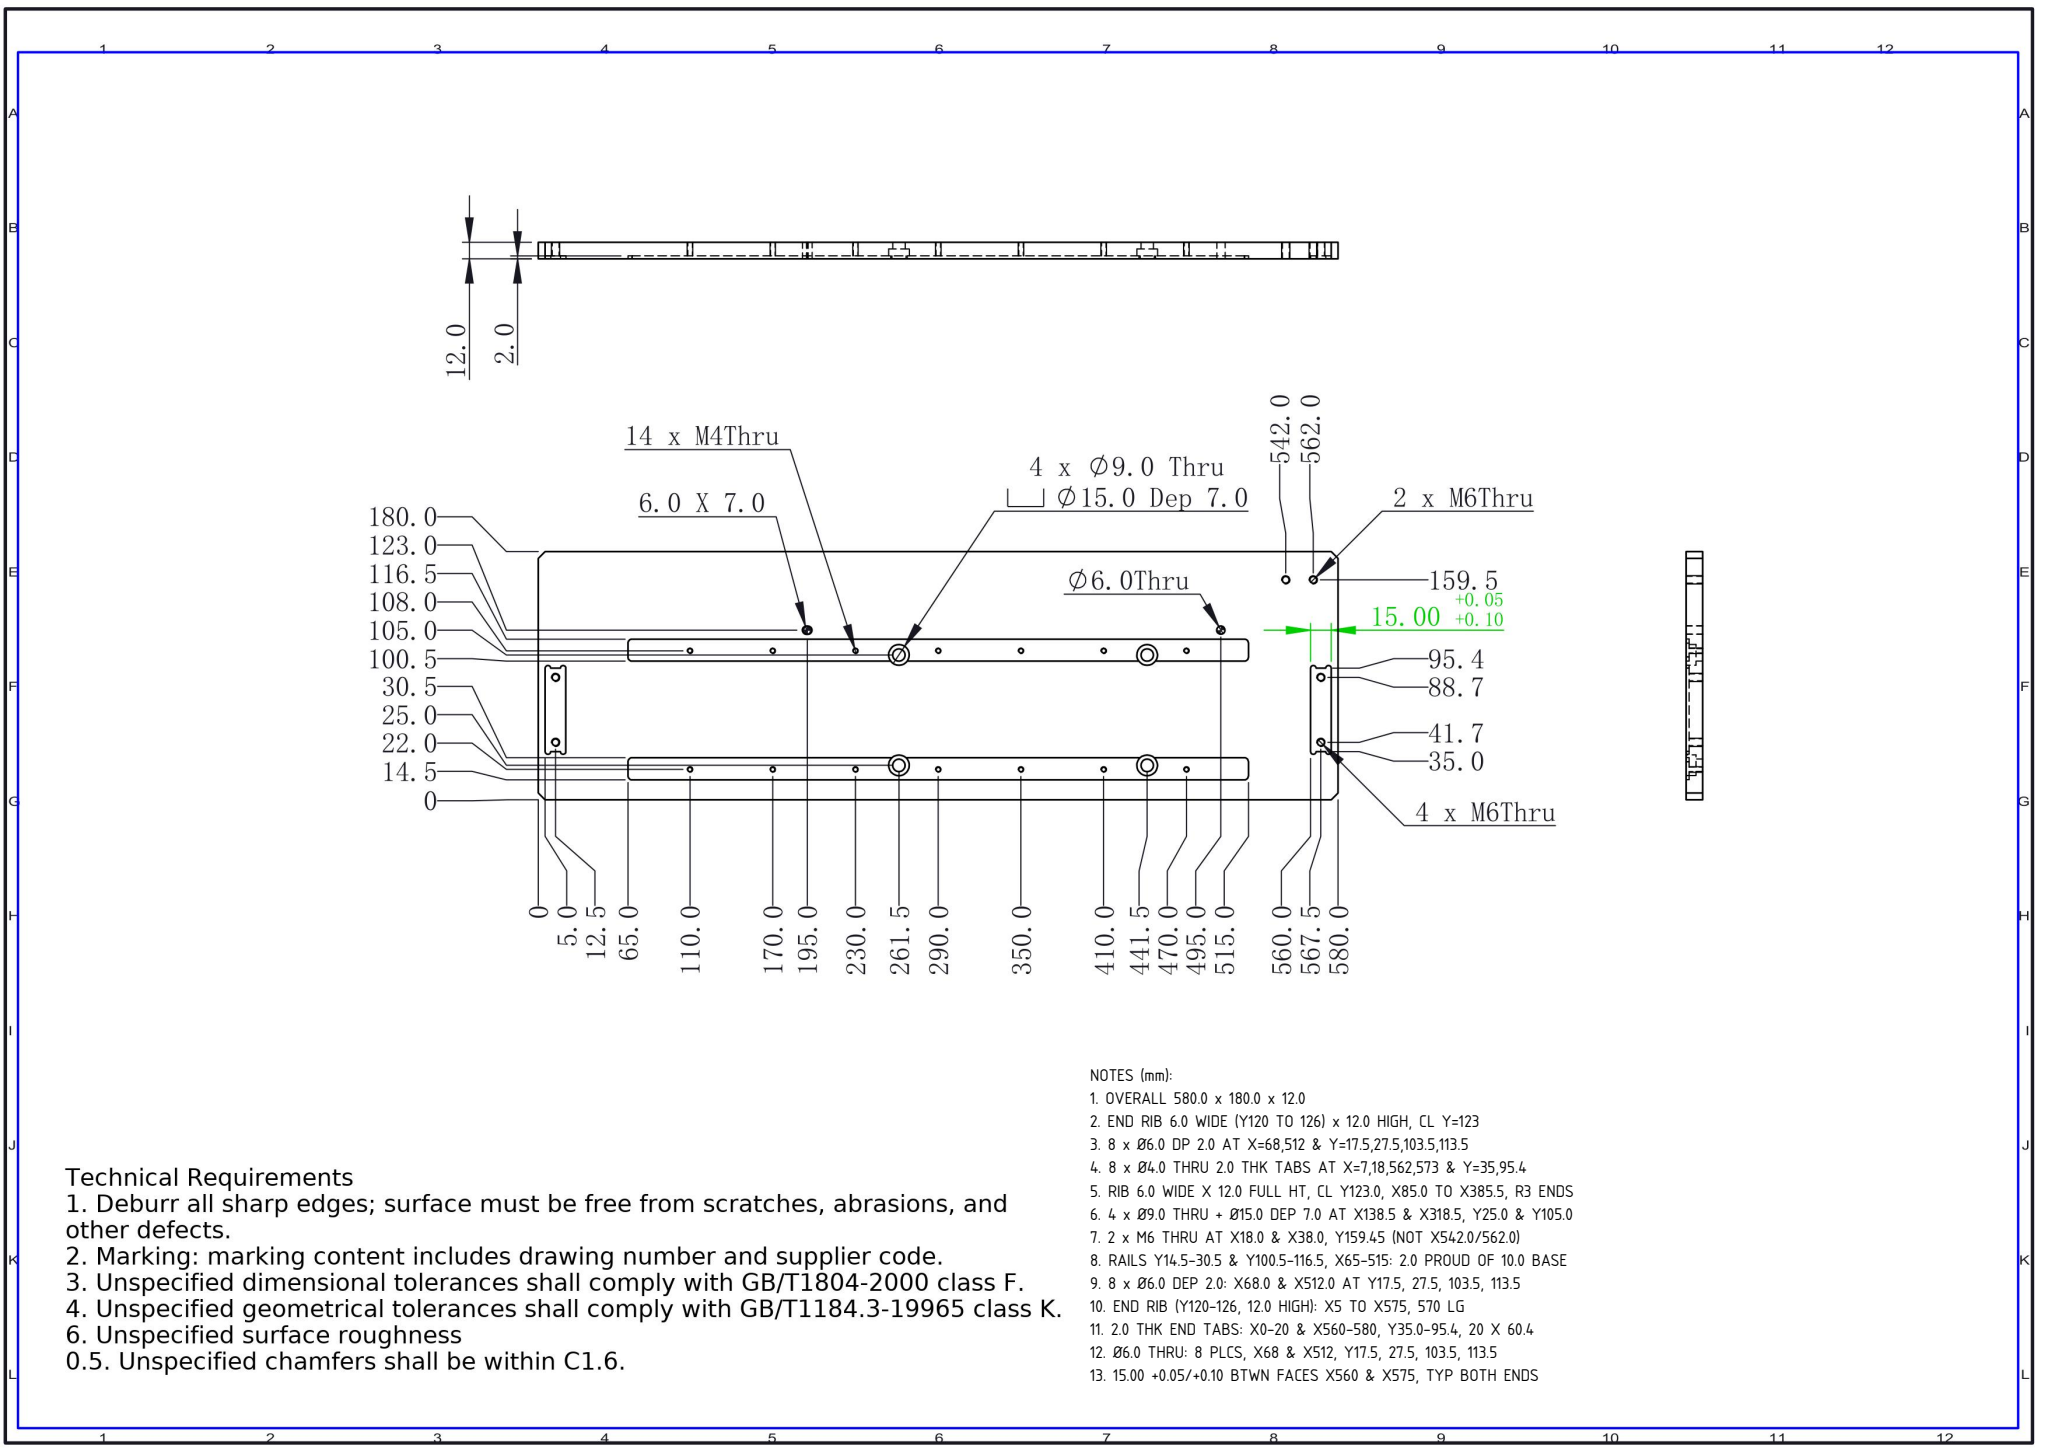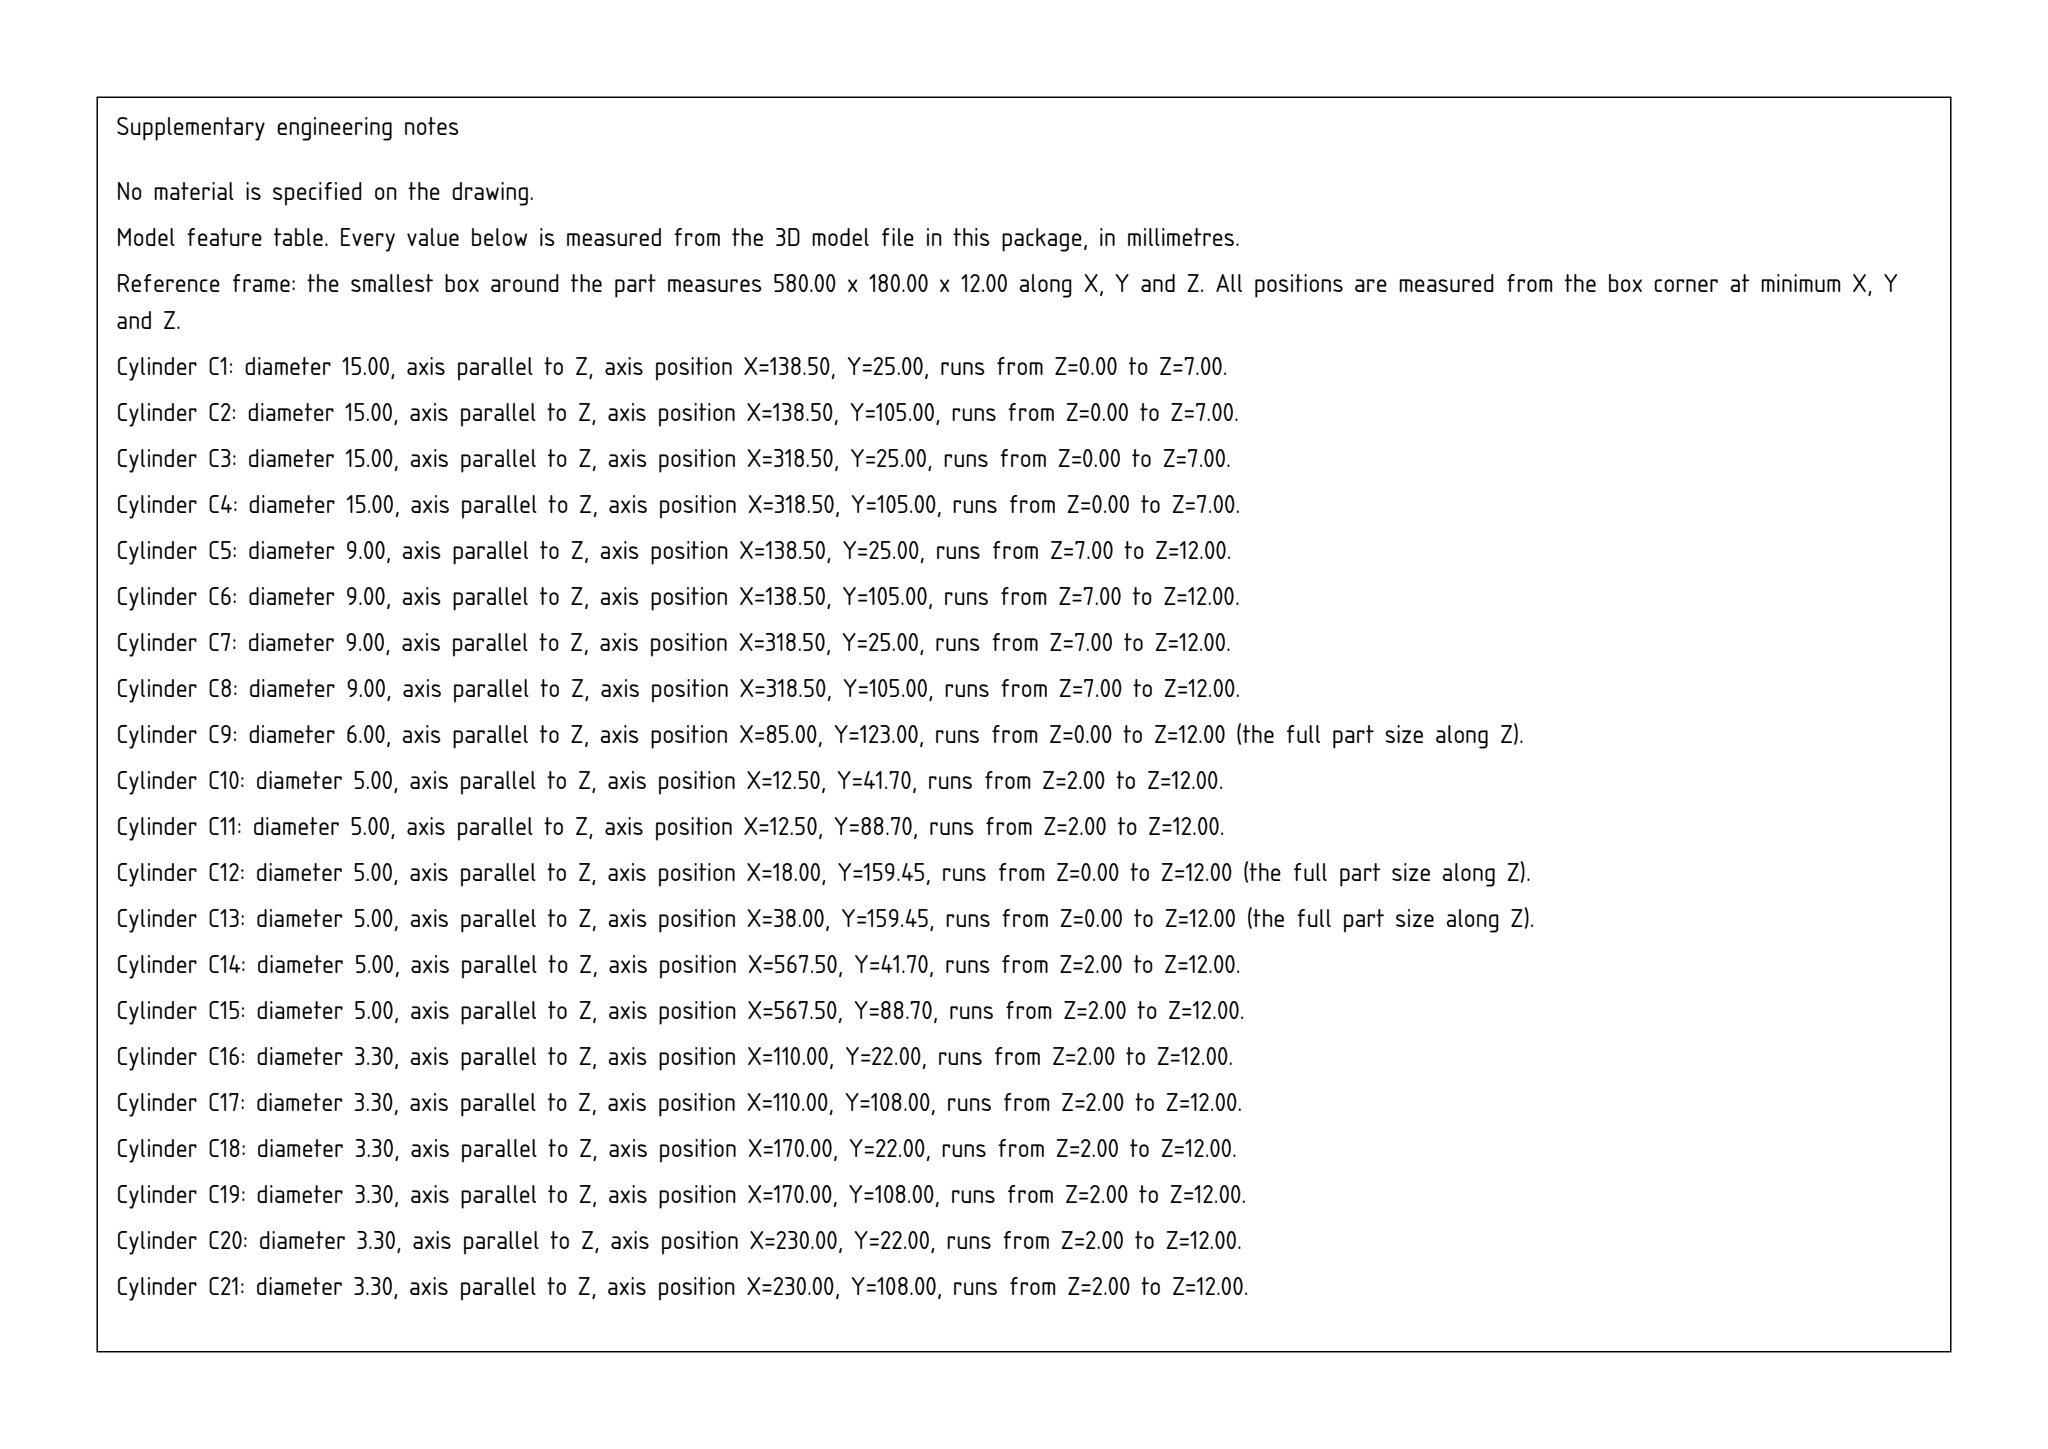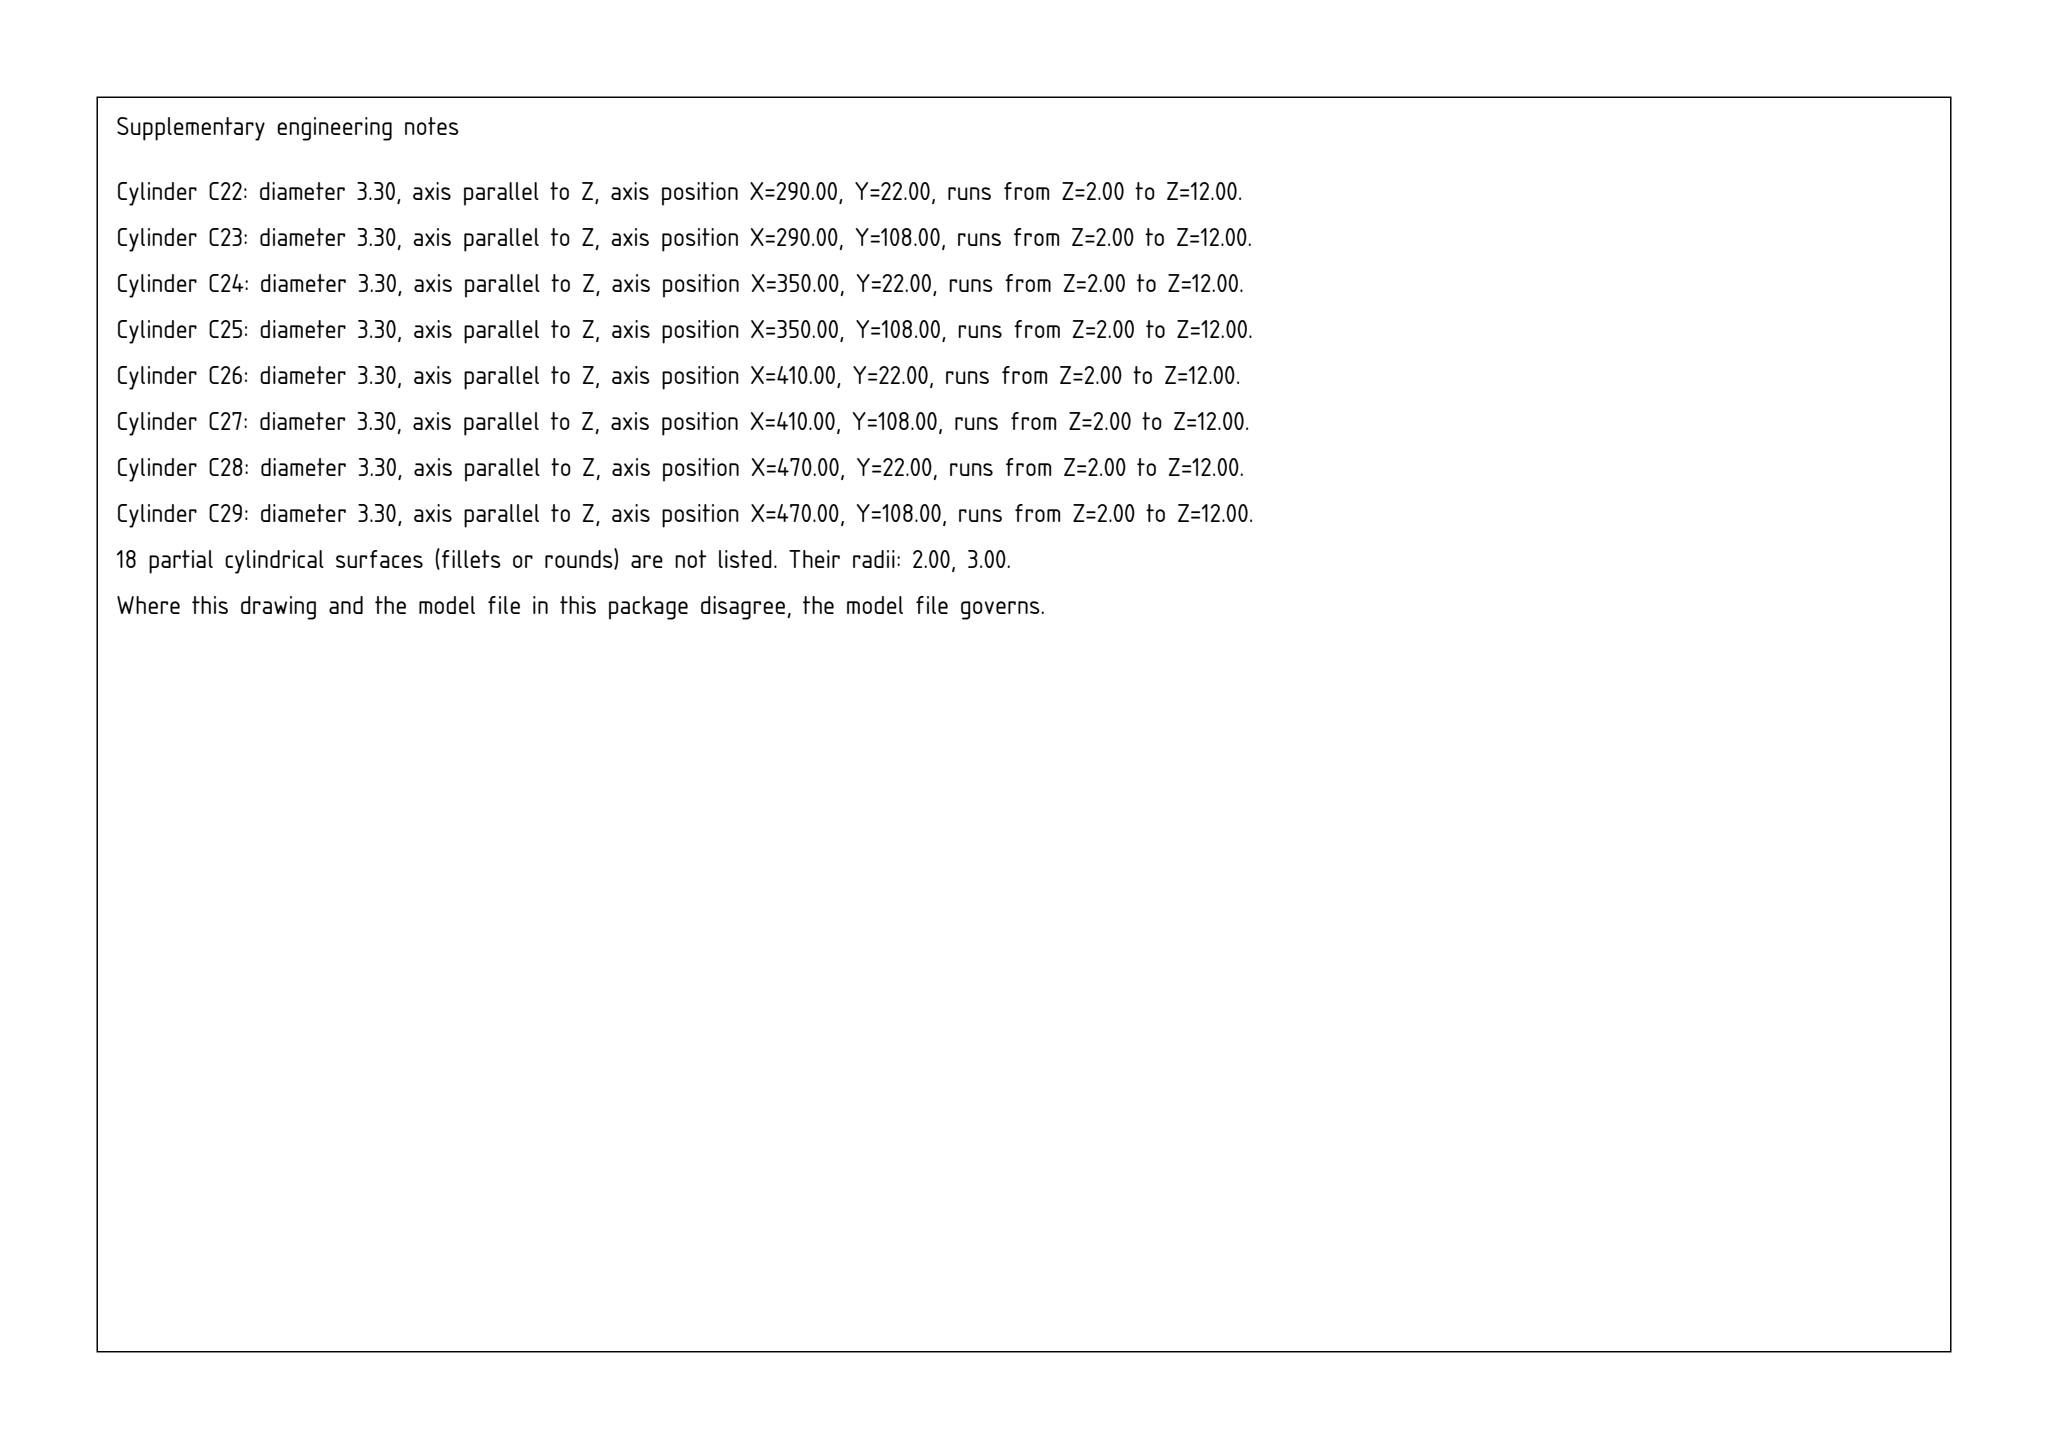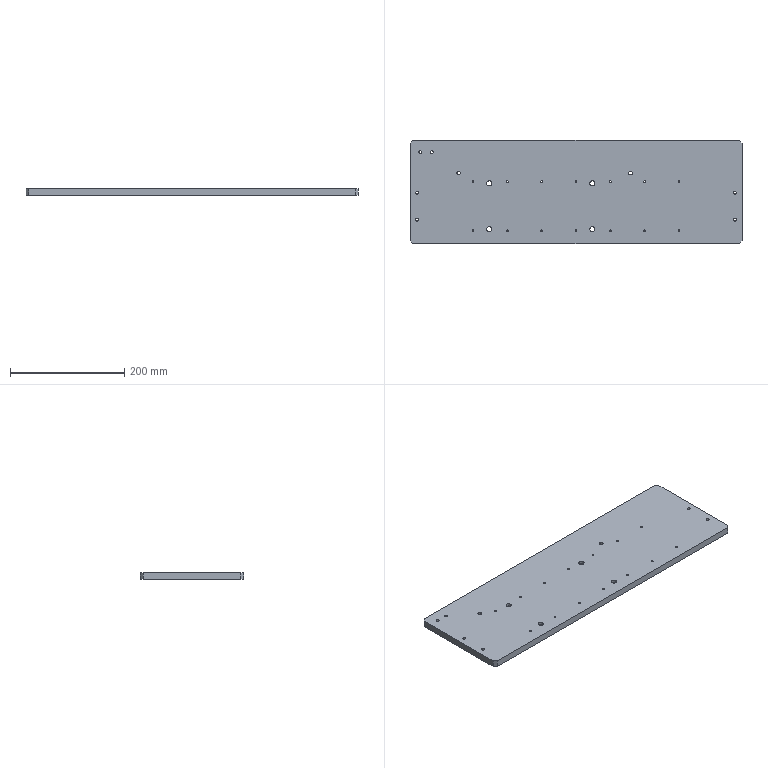Part | SolidWorks | mm | 1 solid | 117 faces | box 580 x 180 x 12 mm | volume 1211538 mm3 | cylinder 77 | plane 40 | commonest cylinder face diameters 3.3 x28 6 x13 5 x12 9 x8 15 x8 4 x8
Drawing notes:
OVERALL 580.0 x 180.0 x 12.0 | from the solid: bbox_xyz 580.0 x 180.0 x 12.0
END RIB 6.0 WIDE (Y120 TO 126) x 12.0 HIGH, CL Y=123 | from the solid: y planes 120 & 126; Ø6 len12 holes at y=123; z planes 0-12
8 x Ø6.0 DP 2.0 AT X=68,512 & Y=17.5,27.5,103.5,113.5 | from the solid: Ø6.0 z-cyls len 2.0 at (68/512, 17.5/27.5/103.5/113.5)
8 x Ø4.0 THRU 2.0 THK TABS AT X=7,18,562,573 & Y=35,95.4 | from the solid: Ø4.0 z-holes len 2.0 at x=7,18,562,573; y=35 & 95.4
RIB 6.0 WIDE X 12.0 FULL HT, CL Y123.0, X85.0 TO X385.5, R3 ENDS | from the solid: Ø6.0 z-cyl len 12.0 at (85.0,123.0) & (384.5/385.5,123.0); y-planes 120.0 & 126.0; bbox z=12.0
4 x Ø9.0 THRU + Ø15.0 DEP 7.0 AT X138.5 & X318.5, Y25.0 & Y105.0 | from the solid: Ø9.0 z-cyl at (138.5,25.0)(138.5,105.0)(318.5,25.0)(318.5,105.0); Ø15.0 len 7.0 same XY
2 x M6 THRU AT X18.0 & X38.0, Y159.45 (NOT X542.0/562.0) | from the solid: Ø5.0 z-cyl len 12.0 at (18.0,159.45) and (38.0,159.45)
RAILS Y14.5-30.5 & Y100.5-116.5, X65-515: 2.0 PROUD OF 10.0 BASE | from the solid: z-planes 0.0/2.0/12.0; x-planes 65.0 & 515.0; y-planes 14.5,30.5,100.5,116.5; M4 cyl len 10.0
8 x Ø6.0 DEP 2.0: X68.0 & X512.0 AT Y17.5, 27.5, 103.5, 113.5 | from the solid: Ø6.0 z-cyl len 2.0 at (68.0 & 512.0) x (17.5, 27.5, 103.5, 113.5)
END RIB (Y120-126, 12.0 HIGH): X5 TO X575, 570 LG | from the solid: axis_planes x=5.0(1) & x=575.0(1) bound rib btwn y-planes 120.0/126.0, z=12.0; rib holes dia6 L12 at y=123
2.0 THK END TABS: X0-20 & X560-580, Y35.0-95.4, 20 X 60.4 | from the solid: x-planes 0.0,20.0,560.0,580.0; y-planes 35.0(2) & 95.4(2); dia4.0 L2.0 holes at (7,35),(7,95.4),(18,35),(18,95.4) mirrored at 562/573
Ø6.0 THRU: 8 PLCS, X68 & X512, Y17.5, 27.5, 103.5, 113.5 | from the solid: dia6.0 z-cyls L2.0 at (68,17.5),(68,27.5),(68,103.5),(68,113.5) and same at x=512
15.00 +0.05/+0.10 BTWN FACES X560 & X575, TYP BOTH ENDS | from the solid: x-planes 5.0 & 20.0 (=575 & 560 in dwg datum) spaced 15.0; one each end
build123d program:
from build123d import *

# Parameters (mm, degrees)
SKETCH1_W                                       = 580
SKETCH1_H                                       = 180
BOSS_EXTRUDE1_DEPTH                             = 12
SKETCH2_W                                       = 15
SKETCH2_H                                       = 60.4
CUT_EXTRUDE1_DEPTH                              = 2
SKETCH3_R                                       = 2
CUT_EXTRUDE3_DEPTH                              = 2
M6_TAPPED_HOLE1_D                               = 5
SKETCH6_W                                       = 450
SKETCH6_H                                       = 16
CUT_EXTRUDE4_DEPTH                              = 2
FILLET1_R                                       = 3
M4_TAPPED_HOLE1_D                               = 3.3
M6_TAPPED_HOLE2_D                               = 5
SIZE_MM_DOWEL_HOLE1_D                           = 6
CUT_EXTRUDE5_DEPTH                              = 304.882
CHAMFER1_SIZE                                   = 5
M8_HEX_SOCKET_HEAD_CAP_SCREW_CBORE1_D           = 9
M8_HEX_SOCKET_HEAD_CAP_SCREW_CBORE1_CBORE_D     = 15
M8_HEX_SOCKET_HEAD_CAP_SCREW_CBORE1_CBORE_DEPTH = 7


with BuildPart() as part:
    # Sketch1 → Boss-Extrude1 (new body)
    with BuildSketch(Plane.XY):
        Rectangle(SKETCH1_W, SKETCH1_H)
    extrude(amount=BOSS_EXTRUDE1_DEPTH)

    # Sketch2 → Cut-Extrude1 (cut)
    with BuildSketch(Plane.XY):
        with Locations((277.5, -24.8)):
            Rectangle(SKETCH2_W, SKETCH2_H)
    cut_extrude1 = extrude(amount=CUT_EXTRUDE1_DEPTH, mode=Mode.SUBTRACT)

    # Sketch3 → Cut-Extrude3 (cut)
    with BuildSketch(Plane(origin=(0, 0, 0), x_dir=(-1, 0, 0), z_dir=(0, 0, -1))):
        with Locations((-283, 5.4)):
            Circle(SKETCH3_R)
        with Locations((-272, 5.4)):
            Circle(SKETCH3_R)
        with Locations((-283, -55)):
            Circle(SKETCH3_R)
        with Locations((-272, -55)):
            Circle(SKETCH3_R)
    cut_extrude3 = extrude(amount=-CUT_EXTRUDE3_DEPTH, mode=Mode.SUBTRACT)

    # Mirror1: Cut-Extrude1, Cut-Extrude3 across plane
    add(cut_extrude1.mirror(Plane(origin=(0, 0, 0), x_dir=(0, 0, 1), z_dir=(1, 0, 0))), mode=Mode.SUBTRACT)
    add(cut_extrude3.mirror(Plane(origin=(0, 0, 0), x_dir=(0, 0, 1), z_dir=(1, 0, 0))), mode=Mode.SUBTRACT)

    # M6 Tapped Hole1 (through all)
    with Locations(Plane(origin=(0, 0, 2), x_dir=(-1, 0, 0), z_dir=(0, 0, -1))):
        with Locations((277.5, -1.3), (277.5, -48.3), (-277.5, -1.3), (-277.5, -48.3)):
            Hole(M6_TAPPED_HOLE1_D / 2)

    # Sketch6 → Cut-Extrude4 (cut)
    with BuildSketch(Plane(origin=(0, 0, 0), x_dir=(-1, 0, 0), z_dir=(0, 0, -1))):
        with Locations((0, -67.5)):
            Rectangle(SKETCH6_W, SKETCH6_H)
        with Locations((0, 18.5)):
            Rectangle(SKETCH6_W, SKETCH6_H)
    extrude(amount=-CUT_EXTRUDE4_DEPTH, mode=Mode.SUBTRACT)

    # Fillet1
    fillet1_edges = [part.edges().sort_by_distance(p)[0] for p in [
        (225, -75.5, 1),
        (225, -59.5, 1),
        (-225, -59.5, 1),
        (-225, -75.5, 1),
        (225, 10.5, 1),
        (225, 26.5, 1),
        (-225, 26.5, 1),
        (-225, 10.5, 1),
    ]]
    fillet(fillet1_edges, radius=FILLET1_R)

    # M4 Tapped Hole1 (through all)
    with Locations(Plane(origin=(0, 0, 2), x_dir=(-1, 0, 0), z_dir=(0, 0, -1))):
        with Locations((180, -68), (120, -68), (60, -68), (0, -68), (-60, -68), (-120, -68), (-180, -68), (-180, 18), (-120, 18), (-60, 18), (0, 18), (60, 18), (120, 18), (180, 18)):
            Hole(M4_TAPPED_HOLE1_D / 2)

    # M6 Tapped Hole2 (through all)
    with Locations(Plane(origin=(0, 0, 0), x_dir=(-1, 0, 0), z_dir=(0, 0, -1))):
        with Locations((272, 69.45), (252, 69.45)):
            Hole(M6_TAPPED_HOLE2_D / 2)

    # Size mm Dowel Hole1 (through all)
    with Locations(Plane(origin=(0, 0, 0), x_dir=(-1, 0, 0), z_dir=(0, 0, -1))):
        with Locations((205, 33)):
            Hole(SIZE_MM_DOWEL_HOLE1_D / 2)

    # Sketch13 → Cut-Extrude5 (cut, through all)
    with BuildSketch(Plane(origin=(0, 0, 0), x_dir=(-1, 0, 0), z_dir=(0, 0, -1))):
        with BuildLine():
            Line((-95.5, 36), (-94.5, 36))
            ThreePointArc((-94.5, 36), (-91.5, 33), (-94.5, 30))
            Line((-94.5, 30), (-95.5, 30))
            ThreePointArc((-95.5, 30), (-98.5, 33), (-95.5, 36))
        make_face()
    extrude(amount=-CUT_EXTRUDE5_DEPTH, mode=Mode.SUBTRACT)

    # Chamfer1
    chamfer1_edges = [part.edges().sort_by_distance(p)[0] for p in [
        (290, -90, 6),
        (-290, -90, 6),
        (-290, 90, 6),
        (290, 90, 6),
    ]]
    chamfer(chamfer1_edges, length=CHAMFER1_SIZE)

    # M8 Hex Socket Head Cap Screw CBORE1 (through all)
    with Locations(Plane(origin=(0, 0, 0), x_dir=(-1, 0, 0), z_dir=(0, 0, -1))):
        with Locations((151.5, 15), (151.5, -65), (-28.5, -65), (-28.5, 15)):
            CounterBoreHole(M8_HEX_SOCKET_HEAD_CAP_SCREW_CBORE1_D / 2, M8_HEX_SOCKET_HEAD_CAP_SCREW_CBORE1_CBORE_D / 2, M8_HEX_SOCKET_HEAD_CAP_SCREW_CBORE1_CBORE_DEPTH)


solid = part.part